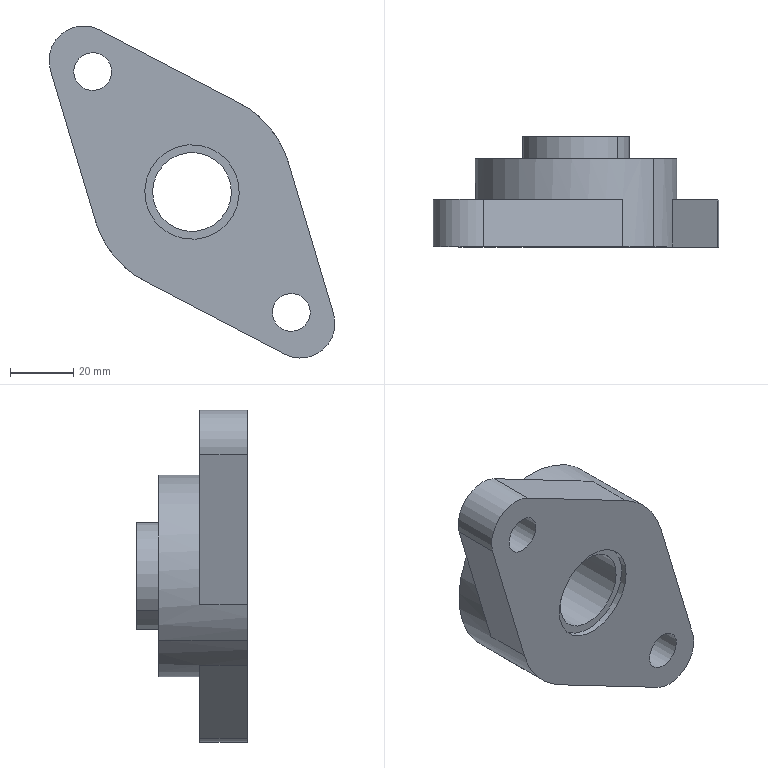Component | SolidWorks | -UCFL205-1 | 1 solid | 24 faces | box 90.73 x 35 x 105.31 mm | volume 107870 mm3 | cylinder 14 | plane 10 | commonest cylinder face diameters 12 x4 30 x2 34 x2 64 x2 25 x2 22 x2
build123d program:
from build123d import *

# Parameters (mm, degrees)
SKETCH1_R           = 6
BOSS_EXTRUDE1_DEPTH = 15
SKETCH2_R           = 32
BOSS_EXTRUDE2_DEPTH = 13
SKETCH3_R           = 12.5
CUT_EXTRUDE1_DEPTH  = 78.672
BOSS_EXTRUDE3_START = 7
SKETCH4_R           = 17
SKETCH4_R_2         = 12.5
BOSS_EXTRUDE3_DEPTH = 7
SKETCH5_R           = 15
CUT_EXTRUDE2_DEPTH  = 2


with BuildPart() as part:
    # Sketch1 → Boss-Extrude1 (new body)
    with BuildSketch(Plane(origin=(0, 0, 0), x_dir=(1, 0, 0), z_dir=(0, 1, 0))):
        with BuildLine():
            Line((-58.278, 10.134), (-12.444, 29.481))
            ThreePointArc((-12.444, 29.481), (0, 32), (12.444, 29.481))
            Line((12.444, 29.481), (58.278, 10.134))
            ThreePointArc((58.278, 10.134), (65, 0), (58.278, -10.134))
            Line((58.278, -10.134), (12.444, -29.481))
            ThreePointArc((12.444, -29.481), (0, -32), (-12.444, -29.481))
            Line((-12.444, -29.481), (-58.278, -10.134))
            ThreePointArc((-58.278, -10.134), (-65, 0), (-58.278, 10.134))
        make_face()
        with Locations(Location((-49.5, 0, 0), (0, 0, 270))):
            Circle(SKETCH1_R, mode=Mode.SUBTRACT)
        with Locations(Location((49.5, 0, 0), (0, 0, 270))):
            Circle(SKETCH1_R, mode=Mode.SUBTRACT)
    extrude(amount=BOSS_EXTRUDE1_DEPTH)

    # Sketch2 → Boss-Extrude2 (add)
    with BuildSketch(Plane(origin=(0, 15, 0), x_dir=(1, 0, 0), z_dir=(0, 1, 0))):
        with Locations(Location((0, 0, 0), (0, 0, 112.885))):
            Circle(SKETCH2_R)
    extrude(amount=BOSS_EXTRUDE2_DEPTH)

    # Sketch3 → Cut-Extrude1 (cut, through all)
    with BuildSketch(Plane(origin=(0, 28, 0), x_dir=(1, 0, 0), z_dir=(0, 1, 0))):
        with Locations(Location((0, 0, 0), (0, 0, 270))):
            Circle(SKETCH3_R)
    extrude(amount=-CUT_EXTRUDE1_DEPTH, mode=Mode.SUBTRACT)

    # Sketch4 → Boss-Extrude3 (add)
    with BuildSketch(Plane(origin=(0, 28, 0), x_dir=(1, 0, 0), z_dir=(0, 1, 0)).offset(BOSS_EXTRUDE3_START)):
        with Locations(Location((0, 0, 0), (0, 0, 270))):
            Circle(SKETCH4_R)
        with Locations(Location((0, 0, 0), (0, 0, 270))):
            Circle(SKETCH4_R_2, mode=Mode.SUBTRACT)
    extrude(amount=-BOSS_EXTRUDE3_DEPTH)

    # Sketch5 → Cut-Extrude2 (cut)
    with BuildSketch(Plane.XZ):
        with Locations(Location((0, 0, 0), (0, 0, 270))):
            Circle(SKETCH5_R)
    extrude(amount=-CUT_EXTRUDE2_DEPTH, mode=Mode.SUBTRACT)


solid = part.part

# Placed as in the assembly
solid = solid.moved(Location((205, 936, -173), (180, -50.479, 180)))
STEP:
#1=COLOUR_RGB('',0.7922,0.8196,0.9333);
#2=FILL_AREA_STYLE_COLOUR('',#1);
#3=FILL_AREA_STYLE('',(#2));
#4=SURFACE_STYLE_FILL_AREA(#3);
#5=SURFACE_SIDE_STYLE('',(#4));
#6=SURFACE_STYLE_USAGE(.BOTH.,#5);
#7=PRESENTATION_STYLE_ASSIGNMENT((#6));
#8=CARTESIAN_POINT('',(8.526,36.929,-6.435));
#9=VERTEX_POINT('',#8);
#10=CARTESIAN_POINT('',(7.615,36.929,-7.187));
#11=VERTEX_POINT('',#10);
#12=CARTESIAN_POINT('',(8.071,36.929,-6.811));
#13=DIRECTION('',(0.,-1.,0.));
#14=DIRECTION('',(-0.7714,0.,-0.6364));
#15=AXIS2_PLACEMENT_3D('',#12,#13,#14);
#16=CIRCLE('',#15,0.5906);
#17=EDGE_CURVE('',#9,#11,#16,.T.);
#18=ORIENTED_EDGE('',*,*,#17,.F.);
#19=CARTESIAN_POINT('',(8.526,36.85,-6.435));
#20=VERTEX_POINT('',#19);
#21=CARTESIAN_POINT('',(8.526,36.929,-6.435));
#22=DIRECTION('',(0.,-1.,0.));
#23=VECTOR('',#22,39.37);
#24=LINE('',#21,#23);
#25=EDGE_CURVE('',#9,#20,#24,.T.);
#26=ORIENTED_EDGE('',*,*,#25,.T.);
#27=CARTESIAN_POINT('',(7.615,36.85,-7.187));
#28=VERTEX_POINT('',#27);
#29=CARTESIAN_POINT('',(8.071,36.85,-6.811));
#30=DIRECTION('',(0.,-1.,0.));
#31=DIRECTION('',(-0.7714,0.,-0.6364));
#32=AXIS2_PLACEMENT_3D('',#29,#30,#31);
#33=CIRCLE('',#32,0.5906);
#34=EDGE_CURVE('',#20,#28,#33,.T.);
#35=ORIENTED_EDGE('',*,*,#34,.T.);
#36=CARTESIAN_POINT('',(7.615,36.929,-7.187));
#37=DIRECTION('',(0.,-1.,0.));
#38=VECTOR('',#37,39.37);
#39=LINE('',#36,#38);
#40=EDGE_CURVE('',#11,#28,#39,.T.);
#41=ORIENTED_EDGE('',*,*,#40,.F.);
#42=EDGE_LOOP('',(#18,#26,#35,#41));
#43=FACE_OUTER_BOUND('',#42,.T.);
#44=CARTESIAN_POINT('',(8.071,36.929,-6.811));
#45=DIRECTION('',(0.,-1.,0.));
#46=DIRECTION('',(-0.7714,0.,-0.6364));
#47=AXIS2_PLACEMENT_3D('',#44,#45,#46);
#48=CYLINDRICAL_SURFACE('',#47,0.5906);
#49=ADVANCED_FACE('',(#43),#48,.F.);
#50=CARTESIAN_POINT('',(8.587,38.228,-6.385));
#51=VERTEX_POINT('',#50);
#52=CARTESIAN_POINT('',(7.555,38.228,-7.237));
#53=VERTEX_POINT('',#52);
#54=CARTESIAN_POINT('',(8.071,38.228,-6.811));
#55=DIRECTION('',(0.,1.,0.));
#56=DIRECTION('',(0.7714,0.,0.6364));
#57=AXIS2_PLACEMENT_3D('',#54,#55,#56);
#58=CIRCLE('',#57,0.6693);
#59=EDGE_CURVE('',#51,#53,#58,.T.);
#60=ORIENTED_EDGE('',*,*,#59,.F.);
#61=CARTESIAN_POINT('',(8.587,37.953,-6.385));
#62=VERTEX_POINT('',#61);
#63=CARTESIAN_POINT('',(8.587,38.228,-6.385));
#64=DIRECTION('',(0.,-1.,0.));
#65=VECTOR('',#64,39.37);
#66=LINE('',#63,#65);
#67=EDGE_CURVE('',#51,#62,#66,.T.);
#68=ORIENTED_EDGE('',*,*,#67,.T.);
#69=CARTESIAN_POINT('',(7.555,37.953,-7.237));
#70=VERTEX_POINT('',#69);
#71=CARTESIAN_POINT('',(8.071,37.953,-6.811));
#72=DIRECTION('',(0.,1.,0.));
#73=DIRECTION('',(0.7714,0.,0.6364));
#74=AXIS2_PLACEMENT_3D('',#71,#72,#73);
#75=CIRCLE('',#74,0.6693);
#76=EDGE_CURVE('',#62,#70,#75,.T.);
#77=ORIENTED_EDGE('',*,*,#76,.T.);
#78=CARTESIAN_POINT('',(7.555,38.228,-7.237));
#79=DIRECTION('',(0.,-1.,0.));
#80=VECTOR('',#79,39.37);
#81=LINE('',#78,#80);
#82=EDGE_CURVE('',#53,#70,#81,.T.);
#83=ORIENTED_EDGE('',*,*,#82,.F.);
#84=EDGE_LOOP('',(#60,#68,#77,#83));
#85=FACE_OUTER_BOUND('',#84,.T.);
#86=CARTESIAN_POINT('',(8.071,38.228,-6.811));
#87=DIRECTION('',(0.,-1.,0.));
#88=DIRECTION('',(-0.7714,0.,-0.6364));
#89=AXIS2_PLACEMENT_3D('',#86,#87,#88);
#90=CYLINDRICAL_SURFACE('',#89,0.6693);
#91=ADVANCED_FACE('',(#85),#90,.T.);
#92=CARTESIAN_POINT('',(9.129,37.441,-8.465));
#93=VERTEX_POINT('',#92);
#94=CARTESIAN_POINT('',(9.493,37.441,-8.164));
#95=VERTEX_POINT('',#94);
#96=CARTESIAN_POINT('',(9.311,37.441,-8.314));
#97=DIRECTION('',(0.,1.,0.));
#98=DIRECTION('',(0.7714,0.,0.6364));
#99=AXIS2_PLACEMENT_3D('',#96,#97,#98);
#100=CIRCLE('',#99,0.2362);
#101=EDGE_CURVE('',#93,#95,#100,.T.);
#102=ORIENTED_EDGE('',*,*,#101,.T.);
#103=CARTESIAN_POINT('',(9.493,36.85,-8.164));
#104=VERTEX_POINT('',#103);
#105=CARTESIAN_POINT('',(9.493,37.441,-8.164));
#106=DIRECTION('',(0.,-1.,0.));
#107=VECTOR('',#106,39.37);
#108=LINE('',#105,#107);
#109=EDGE_CURVE('',#95,#104,#108,.T.);
#110=ORIENTED_EDGE('',*,*,#109,.T.);
#111=CARTESIAN_POINT('',(9.129,36.85,-8.465));
#112=VERTEX_POINT('',#111);
#113=CARTESIAN_POINT('',(9.311,36.85,-8.314));
#114=DIRECTION('',(0.,1.,0.));
#115=DIRECTION('',(0.7714,0.,0.6364));
#116=AXIS2_PLACEMENT_3D('',#113,#114,#115);
#117=CIRCLE('',#116,0.2362);
#118=EDGE_CURVE('',#112,#104,#117,.T.);
#119=ORIENTED_EDGE('',*,*,#118,.F.);
#120=CARTESIAN_POINT('',(9.129,37.441,-8.465));
#121=DIRECTION('',(0.,-1.,0.));
#122=VECTOR('',#121,39.37);
#123=LINE('',#120,#122);
#124=EDGE_CURVE('',#93,#112,#123,.T.);
#125=ORIENTED_EDGE('',*,*,#124,.F.);
#126=EDGE_LOOP('',(#102,#110,#119,#125));
#127=FACE_OUTER_BOUND('',#126,.T.);
#128=CARTESIAN_POINT('',(9.311,37.441,-8.314));
#129=DIRECTION('',(0.,-1.,0.));
#130=DIRECTION('',(-0.7714,0.,-0.6364));
#131=AXIS2_PLACEMENT_3D('',#128,#129,#130);
#132=CYLINDRICAL_SURFACE('',#131,0.2362);
#133=ADVANCED_FACE('',(#127),#132,.F.);
#134=CARTESIAN_POINT('',(6.648,37.441,-5.458));
#135=VERTEX_POINT('',#134);
#136=CARTESIAN_POINT('',(7.013,37.441,-5.157));
#137=VERTEX_POINT('',#136);
#138=CARTESIAN_POINT('',(6.831,37.441,-5.308));
#139=DIRECTION('',(0.,1.,0.));
#140=DIRECTION('',(0.7714,0.,0.6364));
#141=AXIS2_PLACEMENT_3D('',#138,#139,#140);
#142=CIRCLE('',#141,0.2362);
#143=EDGE_CURVE('',#135,#137,#142,.T.);
#144=ORIENTED_EDGE('',*,*,#143,.T.);
#145=CARTESIAN_POINT('',(7.013,36.85,-5.157));
#146=VERTEX_POINT('',#145);
#147=CARTESIAN_POINT('',(7.013,37.441,-5.157));
#148=DIRECTION('',(0.,-1.,0.));
#149=VECTOR('',#148,39.37);
#150=LINE('',#147,#149);
#151=EDGE_CURVE('',#137,#146,#150,.T.);
#152=ORIENTED_EDGE('',*,*,#151,.T.);
#153=CARTESIAN_POINT('',(6.648,36.85,-5.458));
#154=VERTEX_POINT('',#153);
#155=CARTESIAN_POINT('',(6.831,36.85,-5.308));
#156=DIRECTION('',(0.,1.,0.));
#157=DIRECTION('',(0.7714,0.,0.6364));
#158=AXIS2_PLACEMENT_3D('',#155,#156,#157);
#159=CIRCLE('',#158,0.2362);
#160=EDGE_CURVE('',#154,#146,#159,.T.);
#161=ORIENTED_EDGE('',*,*,#160,.F.);
#162=CARTESIAN_POINT('',(6.648,37.441,-5.458));
#163=DIRECTION('',(0.,-1.,0.));
#164=VECTOR('',#163,39.37);
#165=LINE('',#162,#164);
#166=EDGE_CURVE('',#135,#154,#165,.T.);
#167=ORIENTED_EDGE('',*,*,#166,.F.);
#168=EDGE_LOOP('',(#144,#152,#161,#167));
#169=FACE_OUTER_BOUND('',#168,.T.);
#170=CARTESIAN_POINT('',(6.831,37.441,-5.308));
#171=DIRECTION('',(0.,-1.,0.));
#172=DIRECTION('',(-0.7714,0.,-0.6364));
#173=AXIS2_PLACEMENT_3D('',#170,#171,#172);
#174=CYLINDRICAL_SURFACE('',#173,0.2362);
#175=ADVANCED_FACE('',(#169),#174,.F.);
#176=CARTESIAN_POINT('',(9.043,37.953,-6.009));
#177=VERTEX_POINT('',#176);
#178=CARTESIAN_POINT('',(7.099,37.953,-7.613));
#179=VERTEX_POINT('',#178);
#180=CARTESIAN_POINT('',(8.071,37.953,-6.811));
#181=DIRECTION('',(0.,1.,0.));
#182=DIRECTION('',(0.7714,0.,0.6364));
#183=AXIS2_PLACEMENT_3D('',#180,#181,#182);
#184=CIRCLE('',#183,1.26);
#185=EDGE_CURVE('',#177,#179,#184,.T.);
#186=ORIENTED_EDGE('',*,*,#185,.F.);
#187=CARTESIAN_POINT('',(9.043,36.85,-6.009));
#188=VERTEX_POINT('',#187);
#189=CARTESIAN_POINT('',(9.043,37.441,-6.009));
#190=DIRECTION('',(0.,-1.,0.));
#191=VECTOR('',#190,39.37);
#192=LINE('',#189,#191);
#193=EDGE_CURVE('',#177,#188,#192,.T.);
#194=ORIENTED_EDGE('',*,*,#193,.T.);
#195=CARTESIAN_POINT('',(9.278,36.85,-6.45));
#196=VERTEX_POINT('',#195);
#197=CARTESIAN_POINT('',(8.071,36.85,-6.811));
#198=DIRECTION('',(0.,1.,0.));
#199=DIRECTION('',(0.7714,0.,0.6364));
#200=AXIS2_PLACEMENT_3D('',#197,#198,#199);
#201=CIRCLE('',#200,1.26);
#202=EDGE_CURVE('',#188,#196,#201,.T.);
#203=ORIENTED_EDGE('',*,*,#202,.T.);
#204=CARTESIAN_POINT('',(9.278,37.441,-6.45));
#205=VERTEX_POINT('',#204);
#206=CARTESIAN_POINT('',(9.278,37.441,-6.45));
#207=DIRECTION('',(0.,-1.,0.));
#208=VECTOR('',#207,39.37);
#209=LINE('',#206,#208);
#210=EDGE_CURVE('',#205,#196,#209,.T.);
#211=ORIENTED_EDGE('',*,*,#210,.F.);
#212=CARTESIAN_POINT('',(7.487,37.441,-7.928));
#213=VERTEX_POINT('',#212);
#214=CARTESIAN_POINT('',(8.071,37.441,-6.811));
#215=DIRECTION('',(0.,1.,0.));
#216=DIRECTION('',(0.7714,0.,0.6364));
#217=AXIS2_PLACEMENT_3D('',#214,#215,#216);
#218=CIRCLE('',#217,1.26);
#219=EDGE_CURVE('',#205,#213,#218,.T.);
#220=ORIENTED_EDGE('',*,*,#219,.T.);
#221=CARTESIAN_POINT('',(7.487,36.85,-7.928));
#222=VERTEX_POINT('',#221);
#223=CARTESIAN_POINT('',(7.487,37.441,-7.928));
#224=DIRECTION('',(0.,-1.,0.));
#225=VECTOR('',#224,39.37);
#226=LINE('',#223,#225);
#227=EDGE_CURVE('',#213,#222,#226,.T.);
#228=ORIENTED_EDGE('',*,*,#227,.T.);
#229=CARTESIAN_POINT('',(7.099,36.85,-7.613));
#230=VERTEX_POINT('',#229);
#231=CARTESIAN_POINT('',(8.071,36.85,-6.811));
#232=DIRECTION('',(0.,1.,0.));
#233=DIRECTION('',(0.7714,0.,0.6364));
#234=AXIS2_PLACEMENT_3D('',#231,#232,#233);
#235=CIRCLE('',#234,1.26);
#236=EDGE_CURVE('',#222,#230,#235,.T.);
#237=ORIENTED_EDGE('',*,*,#236,.T.);
#238=CARTESIAN_POINT('',(7.099,37.441,-7.613));
#239=DIRECTION('',(0.,-1.,0.));
#240=VECTOR('',#239,39.37);
#241=LINE('',#238,#240);
#242=EDGE_CURVE('',#179,#230,#241,.T.);
#243=ORIENTED_EDGE('',*,*,#242,.F.);
#244=EDGE_LOOP('',(#186,#194,#203,#211,#220,#228,#237,#243));
#245=FACE_OUTER_BOUND('',#244,.T.);
#246=CARTESIAN_POINT('',(8.071,37.441,-6.811));
#247=DIRECTION('',(0.,-1.,0.));
#248=DIRECTION('',(-0.7714,0.,-0.6364));
#249=AXIS2_PLACEMENT_3D('',#246,#247,#248);
#250=CYLINDRICAL_SURFACE('',#249,1.26);
#251=ADVANCED_FACE('',(#245),#250,.T.);
#252=CARTESIAN_POINT('',(7.691,36.929,-7.124));
#253=VERTEX_POINT('',#252);
#254=CARTESIAN_POINT('',(8.45,36.929,-6.498));
#255=VERTEX_POINT('',#254);
#256=CARTESIAN_POINT('',(8.071,36.929,-6.811));
#257=DIRECTION('',(0.,1.,0.));
#258=DIRECTION('',(-0.7714,0.,-0.6364));
#259=AXIS2_PLACEMENT_3D('',#256,#257,#258);
#260=CIRCLE('',#259,0.4921);
#261=EDGE_CURVE('',#253,#255,#260,.T.);
#262=ORIENTED_EDGE('',*,*,#261,.F.);
#263=CARTESIAN_POINT('',(7.691,38.228,-7.124));
#264=VERTEX_POINT('',#263);
#265=CARTESIAN_POINT('',(7.691,36.85,-7.124));
#266=DIRECTION('',(0.,1.,0.));
#267=VECTOR('',#266,39.37);
#268=LINE('',#265,#267);
#269=EDGE_CURVE('',#253,#264,#268,.T.);
#270=ORIENTED_EDGE('',*,*,#269,.T.);
#271=CARTESIAN_POINT('',(8.45,38.228,-6.498));
#272=VERTEX_POINT('',#271);
#273=CARTESIAN_POINT('',(8.071,38.228,-6.811));
#274=DIRECTION('',(0.,1.,0.));
#275=DIRECTION('',(0.7714,0.,0.6364));
#276=AXIS2_PLACEMENT_3D('',#273,#274,#275);
#277=CIRCLE('',#276,0.4921);
#278=EDGE_CURVE('',#264,#272,#277,.T.);
#279=ORIENTED_EDGE('',*,*,#278,.T.);
#280=CARTESIAN_POINT('',(8.45,36.85,-6.498));
#281=DIRECTION('',(0.,1.,0.));
#282=VECTOR('',#281,39.37);
#283=LINE('',#280,#282);
#284=EDGE_CURVE('',#255,#272,#283,.T.);
#285=ORIENTED_EDGE('',*,*,#284,.F.);
#286=EDGE_LOOP('',(#262,#270,#279,#285));
#287=FACE_OUTER_BOUND('',#286,.T.);
#288=CARTESIAN_POINT('',(8.071,36.85,-6.811));
#289=DIRECTION('',(0.,1.,0.));
#290=DIRECTION('',(0.7714,0.,0.6364));
#291=AXIS2_PLACEMENT_3D('',#288,#289,#290);
#292=CYLINDRICAL_SURFACE('',#291,0.4921);
#293=ADVANCED_FACE('',(#287),#292,.F.);
#294=ORIENTED_EDGE('',*,*,#269,.F.);
#295=CARTESIAN_POINT('',(8.071,36.929,-6.811));
#296=DIRECTION('',(0.,1.,0.));
#297=DIRECTION('',(-0.7714,0.,-0.6364));
#298=AXIS2_PLACEMENT_3D('',#295,#296,#297);
#299=CIRCLE('',#298,0.4921);
#300=EDGE_CURVE('',#255,#253,#299,.T.);
#301=ORIENTED_EDGE('',*,*,#300,.F.);
#302=ORIENTED_EDGE('',*,*,#284,.T.);
#303=CARTESIAN_POINT('',(8.071,38.228,-6.811));
#304=DIRECTION('',(0.,1.,0.));
#305=DIRECTION('',(0.7714,0.,0.6364));
#306=AXIS2_PLACEMENT_3D('',#303,#304,#305);
#307=CIRCLE('',#306,0.4921);
#308=EDGE_CURVE('',#272,#264,#307,.T.);
#309=ORIENTED_EDGE('',*,*,#308,.T.);
#310=EDGE_LOOP('',(#294,#301,#302,#309));
#311=FACE_OUTER_BOUND('',#310,.T.);
#312=CARTESIAN_POINT('',(8.071,36.85,-6.811));
#313=DIRECTION('',(0.,1.,0.));
#314=DIRECTION('',(0.7714,0.,0.6364));
#315=AXIS2_PLACEMENT_3D('',#312,#313,#314);
#316=CYLINDRICAL_SURFACE('',#315,0.4921);
#317=ADVANCED_FACE('',(#311),#316,.F.);
#318=CARTESIAN_POINT('',(8.071,37.953,-6.811));
#319=DIRECTION('',(0.,1.,0.));
#320=DIRECTION('',(0.7714,0.,0.6364));
#321=AXIS2_PLACEMENT_3D('',#318,#319,#320);
#322=CIRCLE('',#321,1.26);
#323=EDGE_CURVE('',#179,#177,#322,.T.);
#324=ORIENTED_EDGE('',*,*,#323,.T.);
#325=ORIENTED_EDGE('',*,*,#185,.T.);
#326=EDGE_LOOP('',(#324,#325));
#327=FACE_OUTER_BOUND('',#326,.T.);
#328=CARTESIAN_POINT('',(8.071,37.953,-6.811));
#329=DIRECTION('',(0.,1.,0.));
#330=DIRECTION('',(0.7714,0.,0.6364));
#331=AXIS2_PLACEMENT_3D('',#328,#329,#330);
#332=CIRCLE('',#331,0.6693);
#333=EDGE_CURVE('',#70,#62,#332,.T.);
#334=ORIENTED_EDGE('',*,*,#333,.F.);
#335=ORIENTED_EDGE('',*,*,#76,.F.);
#336=EDGE_LOOP('',(#334,#335));
#337=FACE_BOUND('',#336,.T.);
#338=CARTESIAN_POINT('',(8.071,37.953,-6.811));
#339=DIRECTION('',(0.,1.,0.));
#340=DIRECTION('',(0.7714,0.,0.6364));
#341=AXIS2_PLACEMENT_3D('',#338,#339,#340);
#342=PLANE('',#341);
#343=ADVANCED_FACE('',(#327,#337),#342,.T.);
#344=ORIENTED_EDGE('',*,*,#219,.F.);
#345=CARTESIAN_POINT('',(9.839,37.441,-8.327));
#346=VERTEX_POINT('',#345);
#347=CARTESIAN_POINT('',(9.839,37.441,-8.327));
#348=DIRECTION('',(0.2863,0.,-0.9581));
#349=VECTOR('',#348,39.37);
#350=LINE('',#347,#349);
#351=EDGE_CURVE('',#205,#346,#350,.T.);
#352=ORIENTED_EDGE('',*,*,#351,.T.);
#353=CARTESIAN_POINT('',(9.223,37.441,-8.835));
#354=VERTEX_POINT('',#353);
#355=CARTESIAN_POINT('',(9.424,37.441,-8.451));
#356=DIRECTION('',(0.,1.,0.));
#357=DIRECTION('',(0.7714,0.,0.6364));
#358=AXIS2_PLACEMENT_3D('',#355,#356,#357);
#359=CIRCLE('',#358,0.4331);
#360=EDGE_CURVE('',#346,#354,#359,.T.);
#361=ORIENTED_EDGE('',*,*,#360,.T.);
#362=CARTESIAN_POINT('',(9.223,37.441,-8.835));
#363=DIRECTION('',(-0.8863,0.,0.4632));
#364=VECTOR('',#363,39.37);
#365=LINE('',#362,#364);
#366=EDGE_CURVE('',#354,#213,#365,.T.);
#367=ORIENTED_EDGE('',*,*,#366,.T.);
#368=EDGE_LOOP('',(#344,#352,#361,#367));
#369=FACE_OUTER_BOUND('',#368,.T.);
#370=ORIENTED_EDGE('',*,*,#101,.F.);
#371=CARTESIAN_POINT('',(9.311,37.441,-8.314));
#372=DIRECTION('',(0.,1.,0.));
#373=DIRECTION('',(0.7714,0.,0.6364));
#374=AXIS2_PLACEMENT_3D('',#371,#372,#373);
#375=CIRCLE('',#374,0.2362);
#376=EDGE_CURVE('',#95,#93,#375,.T.);
#377=ORIENTED_EDGE('',*,*,#376,.F.);
#378=EDGE_LOOP('',(#370,#377));
#379=FACE_BOUND('',#378,.T.);
#380=CARTESIAN_POINT('',(6.718,37.441,-5.171));
#381=DIRECTION('',(0.,1.,0.));
#382=DIRECTION('',(0.7714,0.,0.6364));
#383=AXIS2_PLACEMENT_3D('',#380,#381,#382);
#384=PLANE('',#383);
#385=ADVANCED_FACE('',(#369,#379),#384,.T.);
#386=CARTESIAN_POINT('',(6.864,37.441,-7.172));
#387=VERTEX_POINT('',#386);
#388=CARTESIAN_POINT('',(8.654,37.441,-5.694));
#389=VERTEX_POINT('',#388);
#390=CARTESIAN_POINT('',(8.071,37.441,-6.811));
#391=DIRECTION('',(0.,1.,0.));
#392=DIRECTION('',(0.7714,0.,0.6364));
#393=AXIS2_PLACEMENT_3D('',#390,#391,#392);
#394=CIRCLE('',#393,1.26);
#395=EDGE_CURVE('',#387,#389,#394,.T.);
#396=ORIENTED_EDGE('',*,*,#395,.F.);
#397=CARTESIAN_POINT('',(6.303,37.441,-5.295));
#398=VERTEX_POINT('',#397);
#399=CARTESIAN_POINT('',(6.303,37.441,-5.295));
#400=DIRECTION('',(-0.2863,0.,0.9581));
#401=VECTOR('',#400,39.37);
#402=LINE('',#399,#401);
#403=EDGE_CURVE('',#387,#398,#402,.T.);
#404=ORIENTED_EDGE('',*,*,#403,.T.);
#405=CARTESIAN_POINT('',(6.919,37.441,-4.787));
#406=VERTEX_POINT('',#405);
#407=CARTESIAN_POINT('',(6.718,37.441,-5.171));
#408=DIRECTION('',(0.,1.,0.));
#409=DIRECTION('',(0.7714,0.,0.6364));
#410=AXIS2_PLACEMENT_3D('',#407,#408,#409);
#411=CIRCLE('',#410,0.4331);
#412=EDGE_CURVE('',#398,#406,#411,.T.);
#413=ORIENTED_EDGE('',*,*,#412,.T.);
#414=CARTESIAN_POINT('',(6.919,37.441,-4.787));
#415=DIRECTION('',(0.8863,0.,-0.4632));
#416=VECTOR('',#415,39.37);
#417=LINE('',#414,#416);
#418=EDGE_CURVE('',#406,#389,#417,.T.);
#419=ORIENTED_EDGE('',*,*,#418,.T.);
#420=EDGE_LOOP('',(#396,#404,#413,#419));
#421=FACE_OUTER_BOUND('',#420,.T.);
#422=ORIENTED_EDGE('',*,*,#143,.F.);
#423=CARTESIAN_POINT('',(6.831,37.441,-5.308));
#424=DIRECTION('',(0.,1.,0.));
#425=DIRECTION('',(0.7714,0.,0.6364));
#426=AXIS2_PLACEMENT_3D('',#423,#424,#425);
#427=CIRCLE('',#426,0.2362);
#428=EDGE_CURVE('',#137,#135,#427,.T.);
#429=ORIENTED_EDGE('',*,*,#428,.F.);
#430=EDGE_LOOP('',(#422,#429));
#431=FACE_BOUND('',#430,.T.);
#432=CARTESIAN_POINT('',(6.718,37.441,-5.171));
#433=DIRECTION('',(0.,1.,0.));
#434=DIRECTION('',(0.7714,0.,0.6364));
#435=AXIS2_PLACEMENT_3D('',#432,#433,#434);
#436=PLANE('',#435);
#437=ADVANCED_FACE('',(#421,#431),#436,.T.);
#438=CARTESIAN_POINT('',(8.071,36.85,-6.811));
#439=DIRECTION('',(0.,-1.,0.));
#440=DIRECTION('',(-0.7714,0.,-0.6364));
#441=AXIS2_PLACEMENT_3D('',#438,#439,#440);
#442=CIRCLE('',#441,0.5906);
#443=EDGE_CURVE('',#28,#20,#442,.T.);
#444=ORIENTED_EDGE('',*,*,#443,.F.);
#445=ORIENTED_EDGE('',*,*,#34,.F.);
#446=EDGE_LOOP('',(#444,#445));
#447=FACE_BOUND('',#446,.T.);
#448=ORIENTED_EDGE('',*,*,#160,.T.);
#449=CARTESIAN_POINT('',(6.831,36.85,-5.308));
#450=DIRECTION('',(0.,1.,0.));
#451=DIRECTION('',(0.7714,0.,0.6364));
#452=AXIS2_PLACEMENT_3D('',#449,#450,#451);
#453=CIRCLE('',#452,0.2362);
#454=EDGE_CURVE('',#146,#154,#453,.T.);
#455=ORIENTED_EDGE('',*,*,#454,.T.);
#456=EDGE_LOOP('',(#448,#455));
#457=FACE_BOUND('',#456,.T.);
#458=CARTESIAN_POINT('',(6.303,36.85,-5.295));
#459=VERTEX_POINT('',#458);
#460=CARTESIAN_POINT('',(6.919,36.85,-4.787));
#461=VERTEX_POINT('',#460);
#462=CARTESIAN_POINT('',(6.718,36.85,-5.171));
#463=DIRECTION('',(0.,1.,0.));
#464=DIRECTION('',(0.7714,0.,0.6364));
#465=AXIS2_PLACEMENT_3D('',#462,#463,#464);
#466=CIRCLE('',#465,0.4331);
#467=EDGE_CURVE('',#459,#461,#466,.T.);
#468=ORIENTED_EDGE('',*,*,#467,.F.);
#469=CARTESIAN_POINT('',(6.864,36.85,-7.172));
#470=VERTEX_POINT('',#469);
#471=CARTESIAN_POINT('',(6.303,36.85,-5.295));
#472=DIRECTION('',(-0.2863,0.,0.9581));
#473=VECTOR('',#472,39.37);
#474=LINE('',#471,#473);
#475=EDGE_CURVE('',#470,#459,#474,.T.);
#476=ORIENTED_EDGE('',*,*,#475,.F.);
#477=CARTESIAN_POINT('',(8.071,36.85,-6.811));
#478=DIRECTION('',(0.,1.,0.));
#479=DIRECTION('',(0.7714,0.,0.6364));
#480=AXIS2_PLACEMENT_3D('',#477,#478,#479);
#481=CIRCLE('',#480,1.26);
#482=EDGE_CURVE('',#230,#470,#481,.T.);
#483=ORIENTED_EDGE('',*,*,#482,.F.);
#484=ORIENTED_EDGE('',*,*,#236,.F.);
#485=CARTESIAN_POINT('',(9.223,36.85,-8.835));
#486=VERTEX_POINT('',#485);
#487=CARTESIAN_POINT('',(9.223,36.85,-8.835));
#488=DIRECTION('',(-0.8863,0.,0.4632));
#489=VECTOR('',#488,39.37);
#490=LINE('',#487,#489);
#491=EDGE_CURVE('',#486,#222,#490,.T.);
#492=ORIENTED_EDGE('',*,*,#491,.F.);
#493=CARTESIAN_POINT('',(9.839,36.85,-8.327));
#494=VERTEX_POINT('',#493);
#495=CARTESIAN_POINT('',(9.424,36.85,-8.451));
#496=DIRECTION('',(0.,1.,0.));
#497=DIRECTION('',(0.7714,0.,0.6364));
#498=AXIS2_PLACEMENT_3D('',#495,#496,#497);
#499=CIRCLE('',#498,0.4331);
#500=EDGE_CURVE('',#494,#486,#499,.T.);
#501=ORIENTED_EDGE('',*,*,#500,.F.);
#502=CARTESIAN_POINT('',(9.839,36.85,-8.327));
#503=DIRECTION('',(0.2863,0.,-0.9581));
#504=VECTOR('',#503,39.37);
#505=LINE('',#502,#504);
#506=EDGE_CURVE('',#196,#494,#505,.T.);
#507=ORIENTED_EDGE('',*,*,#506,.F.);
#508=ORIENTED_EDGE('',*,*,#202,.F.);
#509=CARTESIAN_POINT('',(8.654,36.85,-5.694));
#510=VERTEX_POINT('',#509);
#511=CARTESIAN_POINT('',(8.071,36.85,-6.811));
#512=DIRECTION('',(0.,1.,0.));
#513=DIRECTION('',(0.7714,0.,0.6364));
#514=AXIS2_PLACEMENT_3D('',#511,#512,#513);
#515=CIRCLE('',#514,1.26);
#516=EDGE_CURVE('',#510,#188,#515,.T.);
#517=ORIENTED_EDGE('',*,*,#516,.F.);
#518=CARTESIAN_POINT('',(6.919,36.85,-4.787));
#519=DIRECTION('',(0.8863,0.,-0.4632));
#520=VECTOR('',#519,39.37);
#521=LINE('',#518,#520);
#522=EDGE_CURVE('',#461,#510,#521,.T.);
#523=ORIENTED_EDGE('',*,*,#522,.F.);
#524=EDGE_LOOP('',(#468,#476,#483,#484,#492,#501,#507,#508,#517,#523));
#525=FACE_OUTER_BOUND('',#524,.T.);
#526=ORIENTED_EDGE('',*,*,#118,.T.);
#527=CARTESIAN_POINT('',(9.311,36.85,-8.314));
#528=DIRECTION('',(0.,1.,0.));
#529=DIRECTION('',(0.7714,0.,0.6364));
#530=AXIS2_PLACEMENT_3D('',#527,#528,#529);
#531=CIRCLE('',#530,0.2362);
#532=EDGE_CURVE('',#104,#112,#531,.T.);
#533=ORIENTED_EDGE('',*,*,#532,.T.);
#534=EDGE_LOOP('',(#526,#533));
#535=FACE_BOUND('',#534,.T.);
#536=CARTESIAN_POINT('',(6.718,36.85,-5.171));
#537=DIRECTION('',(0.,1.,0.));
#538=DIRECTION('',(0.7714,0.,0.6364));
#539=AXIS2_PLACEMENT_3D('',#536,#537,#538);
#540=PLANE('',#539);
#541=ADVANCED_FACE('',(#447,#457,#525,#535),#540,.F.);
#542=ORIENTED_EDGE('',*,*,#467,.T.);
#543=CARTESIAN_POINT('',(6.919,37.441,-4.787));
#544=DIRECTION('',(0.,-1.,0.));
#545=VECTOR('',#544,39.37);
#546=LINE('',#543,#545);
#547=EDGE_CURVE('',#406,#461,#546,.T.);
#548=ORIENTED_EDGE('',*,*,#547,.F.);
#549=ORIENTED_EDGE('',*,*,#412,.F.);
#550=CARTESIAN_POINT('',(6.303,37.441,-5.295));
#551=DIRECTION('',(0.,-1.,0.));
#552=VECTOR('',#551,39.37);
#553=LINE('',#550,#552);
#554=EDGE_CURVE('',#398,#459,#553,.T.);
#555=ORIENTED_EDGE('',*,*,#554,.T.);
#556=EDGE_LOOP('',(#542,#548,#549,#555));
#557=FACE_OUTER_BOUND('',#556,.T.);
#558=CARTESIAN_POINT('',(6.718,37.441,-5.171));
#559=DIRECTION('',(0.,-1.,0.));
#560=DIRECTION('',(-0.7714,0.,-0.6364));
#561=AXIS2_PLACEMENT_3D('',#558,#559,#560);
#562=CYLINDRICAL_SURFACE('',#561,0.4331);
#563=ADVANCED_FACE('',(#557),#562,.T.);
#564=ORIENTED_EDGE('',*,*,#522,.T.);
#565=CARTESIAN_POINT('',(8.654,37.441,-5.694));
#566=DIRECTION('',(0.,-1.,0.));
#567=VECTOR('',#566,39.37);
#568=LINE('',#565,#567);
#569=EDGE_CURVE('',#389,#510,#568,.T.);
#570=ORIENTED_EDGE('',*,*,#569,.F.);
#571=ORIENTED_EDGE('',*,*,#418,.F.);
#572=ORIENTED_EDGE('',*,*,#547,.T.);
#573=EDGE_LOOP('',(#564,#570,#571,#572));
#574=FACE_OUTER_BOUND('',#573,.T.);
#575=CARTESIAN_POINT('',(6.919,37.441,-4.787));
#576=DIRECTION('',(-0.4632,0.,-0.8863));
#577=DIRECTION('',(-0.8863,0.,0.4632));
#578=AXIS2_PLACEMENT_3D('',#575,#576,#577);
#579=PLANE('',#578);
#580=ADVANCED_FACE('',(#574),#579,.F.);
#581=ORIENTED_EDGE('',*,*,#506,.T.);
#582=CARTESIAN_POINT('',(9.839,37.441,-8.327));
#583=DIRECTION('',(0.,-1.,0.));
#584=VECTOR('',#583,39.37);
#585=LINE('',#582,#584);
#586=EDGE_CURVE('',#346,#494,#585,.T.);
#587=ORIENTED_EDGE('',*,*,#586,.F.);
#588=ORIENTED_EDGE('',*,*,#351,.F.);
#589=ORIENTED_EDGE('',*,*,#210,.T.);
#590=EDGE_LOOP('',(#581,#587,#588,#589));
#591=FACE_OUTER_BOUND('',#590,.T.);
#592=CARTESIAN_POINT('',(9.839,37.441,-8.327));
#593=DIRECTION('',(-0.9581,0.,-0.2863));
#594=DIRECTION('',(-0.2863,0.,0.9581));
#595=AXIS2_PLACEMENT_3D('',#592,#593,#594);
#596=PLANE('',#595);
#597=ADVANCED_FACE('',(#591),#596,.F.);
#598=ORIENTED_EDGE('',*,*,#500,.T.);
#599=CARTESIAN_POINT('',(9.223,37.441,-8.835));
#600=DIRECTION('',(0.,-1.,0.));
#601=VECTOR('',#600,39.37);
#602=LINE('',#599,#601);
#603=EDGE_CURVE('',#354,#486,#602,.T.);
#604=ORIENTED_EDGE('',*,*,#603,.F.);
#605=ORIENTED_EDGE('',*,*,#360,.F.);
#606=ORIENTED_EDGE('',*,*,#586,.T.);
#607=EDGE_LOOP('',(#598,#604,#605,#606));
#608=FACE_OUTER_BOUND('',#607,.T.);
#609=CARTESIAN_POINT('',(9.424,37.441,-8.451));
#610=DIRECTION('',(0.,-1.,0.));
#611=DIRECTION('',(-0.7714,0.,-0.6364));
#612=AXIS2_PLACEMENT_3D('',#609,#610,#611);
#613=CYLINDRICAL_SURFACE('',#612,0.4331);
#614=ADVANCED_FACE('',(#608),#613,.T.);
#615=ORIENTED_EDGE('',*,*,#491,.T.);
#616=ORIENTED_EDGE('',*,*,#227,.F.);
#617=ORIENTED_EDGE('',*,*,#366,.F.);
#618=ORIENTED_EDGE('',*,*,#603,.T.);
#619=EDGE_LOOP('',(#615,#616,#617,#618));
#620=FACE_OUTER_BOUND('',#619,.T.);
#621=CARTESIAN_POINT('',(9.223,37.441,-8.835));
#622=DIRECTION('',(0.4632,0.,0.8863));
#623=DIRECTION('',(0.8863,0.,-0.4632));
#624=AXIS2_PLACEMENT_3D('',#621,#622,#623);
#625=PLANE('',#624);
#626=ADVANCED_FACE('',(#620),#625,.F.);
#627=ORIENTED_EDGE('',*,*,#193,.F.);
#628=ORIENTED_EDGE('',*,*,#323,.F.);
#629=ORIENTED_EDGE('',*,*,#242,.T.);
#630=ORIENTED_EDGE('',*,*,#482,.T.);
#631=CARTESIAN_POINT('',(6.864,37.441,-7.172));
#632=DIRECTION('',(0.,-1.,0.));
#633=VECTOR('',#632,39.37);
#634=LINE('',#631,#633);
#635=EDGE_CURVE('',#387,#470,#634,.T.);
#636=ORIENTED_EDGE('',*,*,#635,.F.);
#637=ORIENTED_EDGE('',*,*,#395,.T.);
#638=ORIENTED_EDGE('',*,*,#569,.T.);
#639=ORIENTED_EDGE('',*,*,#516,.T.);
#640=EDGE_LOOP('',(#627,#628,#629,#630,#636,#637,#638,#639));
#641=FACE_OUTER_BOUND('',#640,.T.);
#642=CARTESIAN_POINT('',(8.071,37.441,-6.811));
#643=DIRECTION('',(0.,-1.,0.));
#644=DIRECTION('',(-0.7714,0.,-0.6364));
#645=AXIS2_PLACEMENT_3D('',#642,#643,#644);
#646=CYLINDRICAL_SURFACE('',#645,1.26);
#647=ADVANCED_FACE('',(#641),#646,.T.);
#648=ORIENTED_EDGE('',*,*,#475,.T.);
#649=ORIENTED_EDGE('',*,*,#554,.F.);
#650=ORIENTED_EDGE('',*,*,#403,.F.);
#651=ORIENTED_EDGE('',*,*,#635,.T.);
#652=EDGE_LOOP('',(#648,#649,#650,#651));
#653=FACE_OUTER_BOUND('',#652,.T.);
#654=CARTESIAN_POINT('',(6.303,37.441,-5.295));
#655=DIRECTION('',(0.9581,0.,0.2863));
#656=DIRECTION('',(0.2863,0.,-0.9581));
#657=AXIS2_PLACEMENT_3D('',#654,#655,#656);
#658=PLANE('',#657);
#659=ADVANCED_FACE('',(#653),#658,.F.);
#660=ORIENTED_EDGE('',*,*,#151,.F.);
#661=ORIENTED_EDGE('',*,*,#428,.T.);
#662=ORIENTED_EDGE('',*,*,#166,.T.);
#663=ORIENTED_EDGE('',*,*,#454,.F.);
#664=EDGE_LOOP('',(#660,#661,#662,#663));
#665=FACE_OUTER_BOUND('',#664,.T.);
#666=CARTESIAN_POINT('',(6.831,37.441,-5.308));
#667=DIRECTION('',(0.,-1.,0.));
#668=DIRECTION('',(-0.7714,0.,-0.6364));
#669=AXIS2_PLACEMENT_3D('',#666,#667,#668);
#670=CYLINDRICAL_SURFACE('',#669,0.2362);
#671=ADVANCED_FACE('',(#665),#670,.F.);
#672=ORIENTED_EDGE('',*,*,#109,.F.);
#673=ORIENTED_EDGE('',*,*,#376,.T.);
#674=ORIENTED_EDGE('',*,*,#124,.T.);
#675=ORIENTED_EDGE('',*,*,#532,.F.);
#676=EDGE_LOOP('',(#672,#673,#674,#675));
#677=FACE_OUTER_BOUND('',#676,.T.);
#678=CARTESIAN_POINT('',(9.311,37.441,-8.314));
#679=DIRECTION('',(0.,-1.,0.));
#680=DIRECTION('',(-0.7714,0.,-0.6364));
#681=AXIS2_PLACEMENT_3D('',#678,#679,#680);
#682=CYLINDRICAL_SURFACE('',#681,0.2362);
#683=ADVANCED_FACE('',(#677),#682,.F.);
#684=CARTESIAN_POINT('',(8.071,38.228,-6.811));
#685=DIRECTION('',(0.,1.,0.));
#686=DIRECTION('',(0.7714,0.,0.6364));
#687=AXIS2_PLACEMENT_3D('',#684,#685,#686);
#688=CIRCLE('',#687,0.6693);
#689=EDGE_CURVE('',#53,#51,#688,.T.);
#690=ORIENTED_EDGE('',*,*,#689,.T.);
#691=ORIENTED_EDGE('',*,*,#59,.T.);
#692=EDGE_LOOP('',(#690,#691));
#693=FACE_OUTER_BOUND('',#692,.T.);
#694=ORIENTED_EDGE('',*,*,#308,.F.);
#695=ORIENTED_EDGE('',*,*,#278,.F.);
#696=EDGE_LOOP('',(#694,#695));
#697=FACE_BOUND('',#696,.T.);
#698=CARTESIAN_POINT('',(8.071,38.228,-6.811));
#699=DIRECTION('',(0.,1.,0.));
#700=DIRECTION('',(0.7714,0.,0.6364));
#701=AXIS2_PLACEMENT_3D('',#698,#699,#700);
#702=PLANE('',#701);
#703=ADVANCED_FACE('',(#693,#697),#702,.T.);
#704=ORIENTED_EDGE('',*,*,#67,.F.);
#705=ORIENTED_EDGE('',*,*,#689,.F.);
#706=ORIENTED_EDGE('',*,*,#82,.T.);
#707=ORIENTED_EDGE('',*,*,#333,.T.);
#708=EDGE_LOOP('',(#704,#705,#706,#707));
#709=FACE_OUTER_BOUND('',#708,.T.);
#710=CARTESIAN_POINT('',(8.071,38.228,-6.811));
#711=DIRECTION('',(0.,-1.,0.));
#712=DIRECTION('',(-0.7714,0.,-0.6364));
#713=AXIS2_PLACEMENT_3D('',#710,#711,#712);
#714=CYLINDRICAL_SURFACE('',#713,0.6693);
#715=ADVANCED_FACE('',(#709),#714,.T.);
#716=CARTESIAN_POINT('',(8.071,36.929,-6.811));
#717=DIRECTION('',(0.,-1.,0.));
#718=DIRECTION('',(-0.7714,0.,-0.6364));
#719=AXIS2_PLACEMENT_3D('',#716,#717,#718);
#720=CIRCLE('',#719,0.5906);
#721=EDGE_CURVE('',#11,#9,#720,.T.);
#722=ORIENTED_EDGE('',*,*,#721,.T.);
#723=ORIENTED_EDGE('',*,*,#17,.T.);
#724=EDGE_LOOP('',(#722,#723));
#725=FACE_OUTER_BOUND('',#724,.T.);
#726=ORIENTED_EDGE('',*,*,#300,.T.);
#727=ORIENTED_EDGE('',*,*,#261,.T.);
#728=EDGE_LOOP('',(#726,#727));
#729=FACE_BOUND('',#728,.T.);
#730=CARTESIAN_POINT('',(8.071,36.929,-6.811));
#731=DIRECTION('',(0.,-1.,0.));
#732=DIRECTION('',(-0.7714,0.,-0.6364));
#733=AXIS2_PLACEMENT_3D('',#730,#731,#732);
#734=PLANE('',#733);
#735=ADVANCED_FACE('',(#725,#729),#734,.T.);
#736=ORIENTED_EDGE('',*,*,#25,.F.);
#737=ORIENTED_EDGE('',*,*,#721,.F.);
#738=ORIENTED_EDGE('',*,*,#40,.T.);
#739=ORIENTED_EDGE('',*,*,#443,.T.);
#740=EDGE_LOOP('',(#736,#737,#738,#739));
#741=FACE_OUTER_BOUND('',#740,.T.);
#742=CARTESIAN_POINT('',(8.071,36.929,-6.811));
#743=DIRECTION('',(0.,-1.,0.));
#744=DIRECTION('',(-0.7714,0.,-0.6364));
#745=AXIS2_PLACEMENT_3D('',#742,#743,#744);
#746=CYLINDRICAL_SURFACE('',#745,0.5906);
#747=ADVANCED_FACE('',(#741),#746,.F.);
#748=CLOSED_SHELL('',(#49,#91,#133,#175,#251,#293,#317,#343,#385,#437,#541,#563,#580,#597,#614,#626,#647,#659,#671,#683,#703,#715,#735,#747));
#749=MANIFOLD_SOLID_BREP('',#748);
#750=STYLED_ITEM('',(#7),#749);
#751=PRESENTATION_LAYER_ASSIGNMENT('','',(#750));
#752=(LENGTH_UNIT()NAMED_UNIT(*)SI_UNIT($,.METRE.));
#753=LENGTH_MEASURE_WITH_UNIT(LENGTH_MEASURE(0.0254),#752);
#754=DIMENSIONAL_EXPONENTS(1.,0.,0.,0.,0.,0.,0.);
#755=(CONVERSION_BASED_UNIT('',#753)LENGTH_UNIT()NAMED_UNIT(#754));
#756=UNCERTAINTY_MEASURE_WITH_UNIT(LENGTH_MEASURE(0.00001),#755,'','');
#757=(NAMED_UNIT(*)PLANE_ANGLE_UNIT()SI_UNIT($,.RADIAN.));
#758=(NAMED_UNIT(*)SI_UNIT($,.STERADIAN.)SOLID_ANGLE_UNIT());
#759=(GEOMETRIC_REPRESENTATION_CONTEXT(3)GLOBAL_UNCERTAINTY_ASSIGNED_CONTEXT((#756))GLOBAL_UNIT_ASSIGNED_CONTEXT((#755,#757,#758))REPRESENTATION_CONTEXT('',''));
#760=MECHANICAL_DESIGN_GEOMETRIC_PRESENTATION_REPRESENTATION('',(#750),#759);
#761=CARTESIAN_POINT('',(0.,0.,0.));
#762=DIRECTION('',(0.,0.,1.));
#763=DIRECTION('',(1.,0.,0.));
#764=AXIS2_PLACEMENT_3D('',#761,#762,#763);
#765=(LENGTH_UNIT()NAMED_UNIT(*)SI_UNIT($,.METRE.));
#766=LENGTH_MEASURE_WITH_UNIT(LENGTH_MEASURE(0.0254),#765);
#767=DIMENSIONAL_EXPONENTS(1.,0.,0.,0.,0.,0.,0.);
#768=(CONVERSION_BASED_UNIT('',#766)LENGTH_UNIT()NAMED_UNIT(#767));
#769=UNCERTAINTY_MEASURE_WITH_UNIT(LENGTH_MEASURE(0.00001),#768,'','');
#770=(NAMED_UNIT(*)PLANE_ANGLE_UNIT()SI_UNIT($,.RADIAN.));
#771=(NAMED_UNIT(*)SI_UNIT($,.STERADIAN.)SOLID_ANGLE_UNIT());
#772=(GEOMETRIC_REPRESENTATION_CONTEXT(3)GLOBAL_UNCERTAINTY_ASSIGNED_CONTEXT((#769))GLOBAL_UNIT_ASSIGNED_CONTEXT((#768,#770,#771))REPRESENTATION_CONTEXT('',''));
#773=ADVANCED_BREP_SHAPE_REPRESENTATION('',(#749,#764),#772);